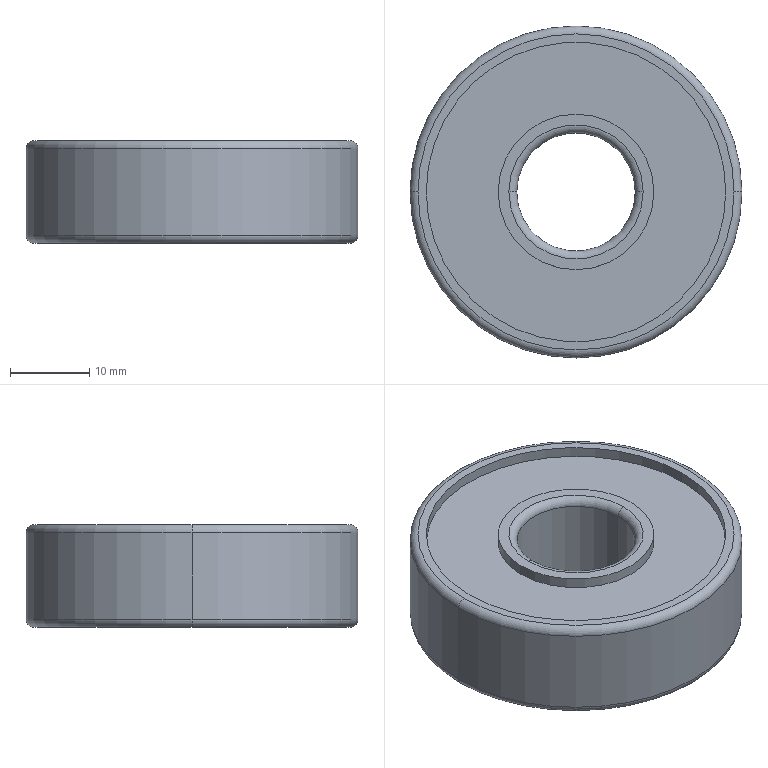Component | SolidWorks | Roller-01-2-1_B6302ZZ-2-1 | 1 solid | 26 faces | box 42 x 42 x 13 mm | volume 13427 mm3 | cylinder 12 | torus 8 | plane 6 | commonest cylinder face diameters 37.9 x4 19.7 x4 42 x2 15 x2
build123d program:
from build123d import *


with BuildPart() as part:
    # Sketch1 → Revolve1 (revolve)
    with BuildSketch(Plane.XY, mode=Mode.PRIVATE) as revolve1_sk:
        with BuildLine():
            Line((0, 20), (0, 18.95))
            Line((0, 18.95), (1.342, 18.95))
            Line((1.342, 18.95), (1.342, 9.85))
            Line((1.342, 9.85), (0, 9.85))
            Line((0, 9.85), (0, 8.5))
            ThreePointArc((0, 8.5), (0.2929, 7.793), (1, 7.5))
            Line((1, 7.5), (12, 7.5))
            ThreePointArc((12, 7.5), (12.707, 7.793), (13, 8.5))
            Line((13, 8.5), (13, 9.85))
            Line((13, 9.85), (11.658, 9.85))
            Line((11.658, 9.85), (11.658, 18.95))
            Line((11.658, 18.95), (13, 18.95))
            Line((13, 18.95), (13, 20))
            ThreePointArc((13, 20), (12.707, 20.707), (12, 21))
            Line((12, 21), (1, 21))
            ThreePointArc((1, 21), (0.2929, 20.707), (0, 20))
        make_face()
    revolve(revolve1_sk.sketch.rotate(Axis((13, 0, 0), (-1, 0, 0)), 270), axis=Axis((13, 0, 0), (-1, 0, 0)))


solid = part.part

# Placed as in the assembly
solid = solid.moved(Location((444.783, 71.385, -23.5), (0, 90, 0)))
STEP:
#1=COLOUR_RGB('',0.7922,0.8196,0.9333);
#2=FILL_AREA_STYLE_COLOUR('',#1);
#3=FILL_AREA_STYLE('',(#2));
#4=SURFACE_STYLE_FILL_AREA(#3);
#5=SURFACE_SIDE_STYLE('',(#4));
#6=SURFACE_STYLE_USAGE(.BOTH.,#5);
#7=PRESENTATION_STYLE_ASSIGNMENT((#6));
#8=CARTESIAN_POINT('',(18.338,2.81,-1.398));
#9=VERTEX_POINT('',#8);
#10=CARTESIAN_POINT('',(16.684,2.81,-1.398));
#11=VERTEX_POINT('',#10);
#12=CARTESIAN_POINT('',(17.511,2.81,-1.398));
#13=DIRECTION('',(0.,0.,1.));
#14=DIRECTION('',(1.,0.,0.));
#15=AXIS2_PLACEMENT_3D('',#12,#13,#14);
#16=CIRCLE('',#15,0.8268);
#17=EDGE_CURVE('',#9,#11,#16,.T.);
#18=ORIENTED_EDGE('',*,*,#17,.T.);
#19=CARTESIAN_POINT('',(16.684,2.81,-0.9646));
#20=VERTEX_POINT('',#19);
#21=CARTESIAN_POINT('',(16.684,2.81,-1.437));
#22=DIRECTION('',(0.,0.,1.));
#23=VECTOR('',#22,39.37);
#24=LINE('',#21,#23);
#25=EDGE_CURVE('',#11,#20,#24,.T.);
#26=ORIENTED_EDGE('',*,*,#25,.T.);
#27=CARTESIAN_POINT('',(18.338,2.81,-0.9646));
#28=VERTEX_POINT('',#27);
#29=CARTESIAN_POINT('',(17.511,2.81,-0.9646));
#30=DIRECTION('',(0.,0.,1.));
#31=DIRECTION('',(1.,0.,0.));
#32=AXIS2_PLACEMENT_3D('',#29,#30,#31);
#33=CIRCLE('',#32,0.8268);
#34=EDGE_CURVE('',#28,#20,#33,.T.);
#35=ORIENTED_EDGE('',*,*,#34,.F.);
#36=CARTESIAN_POINT('',(18.338,2.81,-1.437));
#37=DIRECTION('',(0.,0.,1.));
#38=VECTOR('',#37,39.37);
#39=LINE('',#36,#38);
#40=EDGE_CURVE('',#9,#28,#39,.T.);
#41=ORIENTED_EDGE('',*,*,#40,.F.);
#42=EDGE_LOOP('',(#18,#26,#35,#41));
#43=FACE_OUTER_BOUND('',#42,.T.);
#44=CARTESIAN_POINT('',(17.511,2.81,-1.437));
#45=DIRECTION('',(0.,0.,1.));
#46=DIRECTION('',(1.,0.,0.));
#47=AXIS2_PLACEMENT_3D('',#44,#45,#46);
#48=CYLINDRICAL_SURFACE('',#47,0.8268);
#49=ADVANCED_FACE('',(#43),#48,.T.);
#50=CARTESIAN_POINT('',(18.299,2.81,-1.437));
#51=VERTEX_POINT('',#50);
#52=CARTESIAN_POINT('',(16.724,2.81,-1.437));
#53=VERTEX_POINT('',#52);
#54=CARTESIAN_POINT('',(17.511,2.81,-1.437));
#55=DIRECTION('',(0.,0.,1.));
#56=DIRECTION('',(1.,0.,0.));
#57=AXIS2_PLACEMENT_3D('',#54,#55,#56);
#58=CIRCLE('',#57,0.7874);
#59=EDGE_CURVE('',#51,#53,#58,.T.);
#60=ORIENTED_EDGE('',*,*,#59,.T.);
#61=CARTESIAN_POINT('',(16.724,2.81,-1.398));
#62=DIRECTION('',(0.,1.,0.));
#63=DIRECTION('',(-1.,0.,0.));
#64=AXIS2_PLACEMENT_3D('',#61,#62,#63);
#65=CIRCLE('',#64,0.03937);
#66=EDGE_CURVE('',#53,#11,#65,.T.);
#67=ORIENTED_EDGE('',*,*,#66,.T.);
#68=ORIENTED_EDGE('',*,*,#17,.F.);
#69=CARTESIAN_POINT('',(18.299,2.81,-1.398));
#70=DIRECTION('',(0.,-1.,0.));
#71=DIRECTION('',(0.,0.,-1.));
#72=AXIS2_PLACEMENT_3D('',#69,#70,#71);
#73=CIRCLE('',#72,0.03937);
#74=EDGE_CURVE('',#51,#9,#73,.T.);
#75=ORIENTED_EDGE('',*,*,#74,.F.);
#76=EDGE_LOOP('',(#60,#67,#68,#75));
#77=FACE_OUTER_BOUND('',#76,.T.);
#78=CARTESIAN_POINT('',(17.511,2.81,-1.398));
#79=DIRECTION('',(0.,0.,1.));
#80=DIRECTION('',(1.,0.,0.));
#81=AXIS2_PLACEMENT_3D('',#78,#79,#80);
#82=TOROIDAL_SURFACE('',#81,0.7874,0.03937);
#83=ADVANCED_FACE('',(#77),#82,.T.);
#84=CARTESIAN_POINT('',(16.765,2.81,-1.437));
#85=VERTEX_POINT('',#84);
#86=CARTESIAN_POINT('',(18.257,2.81,-1.437));
#87=VERTEX_POINT('',#86);
#88=CARTESIAN_POINT('',(17.511,2.81,-1.437));
#89=DIRECTION('',(0.,0.,1.));
#90=DIRECTION('',(1.,0.,0.));
#91=AXIS2_PLACEMENT_3D('',#88,#89,#90);
#92=CIRCLE('',#91,0.7461);
#93=EDGE_CURVE('',#85,#87,#92,.T.);
#94=ORIENTED_EDGE('',*,*,#93,.F.);
#95=CARTESIAN_POINT('',(16.765,2.81,-1.384));
#96=VERTEX_POINT('',#95);
#97=CARTESIAN_POINT('',(16.765,2.81,-1.437));
#98=DIRECTION('',(0.,0.,1.));
#99=VECTOR('',#98,39.37);
#100=LINE('',#97,#99);
#101=EDGE_CURVE('',#85,#96,#100,.T.);
#102=ORIENTED_EDGE('',*,*,#101,.T.);
#103=CARTESIAN_POINT('',(18.257,2.81,-1.384));
#104=VERTEX_POINT('',#103);
#105=CARTESIAN_POINT('',(17.511,2.81,-1.384));
#106=DIRECTION('',(0.,0.,1.));
#107=DIRECTION('',(1.,0.,0.));
#108=AXIS2_PLACEMENT_3D('',#105,#106,#107);
#109=CIRCLE('',#108,0.7461);
#110=EDGE_CURVE('',#96,#104,#109,.T.);
#111=ORIENTED_EDGE('',*,*,#110,.T.);
#112=CARTESIAN_POINT('',(18.257,2.81,-1.437));
#113=DIRECTION('',(0.,0.,1.));
#114=VECTOR('',#113,39.37);
#115=LINE('',#112,#114);
#116=EDGE_CURVE('',#87,#104,#115,.T.);
#117=ORIENTED_EDGE('',*,*,#116,.F.);
#118=EDGE_LOOP('',(#94,#102,#111,#117));
#119=FACE_OUTER_BOUND('',#118,.T.);
#120=CARTESIAN_POINT('',(17.511,2.81,-1.437));
#121=DIRECTION('',(0.,0.,1.));
#122=DIRECTION('',(1.,0.,0.));
#123=AXIS2_PLACEMENT_3D('',#120,#121,#122);
#124=CYLINDRICAL_SURFACE('',#123,0.7461);
#125=ADVANCED_FACE('',(#119),#124,.F.);
#126=CARTESIAN_POINT('',(17.899,2.81,-1.437));
#127=VERTEX_POINT('',#126);
#128=CARTESIAN_POINT('',(17.123,2.81,-1.437));
#129=VERTEX_POINT('',#128);
#130=CARTESIAN_POINT('',(17.511,2.81,-1.437));
#131=DIRECTION('',(0.,0.,1.));
#132=DIRECTION('',(1.,0.,0.));
#133=AXIS2_PLACEMENT_3D('',#130,#131,#132);
#134=CIRCLE('',#133,0.3878);
#135=EDGE_CURVE('',#127,#129,#134,.T.);
#136=ORIENTED_EDGE('',*,*,#135,.T.);
#137=CARTESIAN_POINT('',(17.123,2.81,-1.384));
#138=VERTEX_POINT('',#137);
#139=CARTESIAN_POINT('',(17.123,2.81,-1.437));
#140=DIRECTION('',(0.,0.,1.));
#141=VECTOR('',#140,39.37);
#142=LINE('',#139,#141);
#143=EDGE_CURVE('',#129,#138,#142,.T.);
#144=ORIENTED_EDGE('',*,*,#143,.T.);
#145=CARTESIAN_POINT('',(17.899,2.81,-1.384));
#146=VERTEX_POINT('',#145);
#147=CARTESIAN_POINT('',(17.511,2.81,-1.384));
#148=DIRECTION('',(0.,0.,1.));
#149=DIRECTION('',(1.,0.,0.));
#150=AXIS2_PLACEMENT_3D('',#147,#148,#149);
#151=CIRCLE('',#150,0.3878);
#152=EDGE_CURVE('',#146,#138,#151,.T.);
#153=ORIENTED_EDGE('',*,*,#152,.F.);
#154=CARTESIAN_POINT('',(17.899,2.81,-1.437));
#155=DIRECTION('',(0.,0.,1.));
#156=VECTOR('',#155,39.37);
#157=LINE('',#154,#156);
#158=EDGE_CURVE('',#127,#146,#157,.T.);
#159=ORIENTED_EDGE('',*,*,#158,.F.);
#160=EDGE_LOOP('',(#136,#144,#153,#159));
#161=FACE_OUTER_BOUND('',#160,.T.);
#162=CARTESIAN_POINT('',(17.511,2.81,-1.437));
#163=DIRECTION('',(0.,0.,1.));
#164=DIRECTION('',(1.,0.,0.));
#165=AXIS2_PLACEMENT_3D('',#162,#163,#164);
#166=CYLINDRICAL_SURFACE('',#165,0.3878);
#167=ADVANCED_FACE('',(#161),#166,.T.);
#168=CARTESIAN_POINT('',(17.806,2.81,-1.398));
#169=VERTEX_POINT('',#168);
#170=CARTESIAN_POINT('',(17.216,2.81,-1.398));
#171=VERTEX_POINT('',#170);
#172=CARTESIAN_POINT('',(17.511,2.81,-1.398));
#173=DIRECTION('',(0.,0.,1.));
#174=DIRECTION('',(1.,0.,0.));
#175=AXIS2_PLACEMENT_3D('',#172,#173,#174);
#176=CIRCLE('',#175,0.2953);
#177=EDGE_CURVE('',#169,#171,#176,.T.);
#178=ORIENTED_EDGE('',*,*,#177,.T.);
#179=CARTESIAN_POINT('',(17.177,2.81,-1.437));
#180=VERTEX_POINT('',#179);
#181=CARTESIAN_POINT('',(17.177,2.81,-1.398));
#182=DIRECTION('',(0.,1.,0.));
#183=DIRECTION('',(-1.,0.,0.));
#184=AXIS2_PLACEMENT_3D('',#181,#182,#183);
#185=CIRCLE('',#184,0.03937);
#186=EDGE_CURVE('',#171,#180,#185,.T.);
#187=ORIENTED_EDGE('',*,*,#186,.T.);
#188=CARTESIAN_POINT('',(17.846,2.81,-1.437));
#189=VERTEX_POINT('',#188);
#190=CARTESIAN_POINT('',(17.511,2.81,-1.437));
#191=DIRECTION('',(0.,0.,1.));
#192=DIRECTION('',(1.,0.,0.));
#193=AXIS2_PLACEMENT_3D('',#190,#191,#192);
#194=CIRCLE('',#193,0.3346);
#195=EDGE_CURVE('',#189,#180,#194,.T.);
#196=ORIENTED_EDGE('',*,*,#195,.F.);
#197=CARTESIAN_POINT('',(17.846,2.81,-1.398));
#198=DIRECTION('',(0.,-1.,0.));
#199=DIRECTION('',(0.,0.,-1.));
#200=AXIS2_PLACEMENT_3D('',#197,#198,#199);
#201=CIRCLE('',#200,0.03937);
#202=EDGE_CURVE('',#169,#189,#201,.T.);
#203=ORIENTED_EDGE('',*,*,#202,.F.);
#204=EDGE_LOOP('',(#178,#187,#196,#203));
#205=FACE_OUTER_BOUND('',#204,.T.);
#206=CARTESIAN_POINT('',(17.511,2.81,-1.398));
#207=DIRECTION('',(0.,0.,1.));
#208=DIRECTION('',(1.,0.,0.));
#209=AXIS2_PLACEMENT_3D('',#206,#207,#208);
#210=TOROIDAL_SURFACE('',#209,0.3346,0.03937);
#211=ADVANCED_FACE('',(#205),#210,.T.);
#212=CARTESIAN_POINT('',(17.511,2.81,-1.398));
#213=DIRECTION('',(0.,0.,1.));
#214=DIRECTION('',(1.,0.,0.));
#215=AXIS2_PLACEMENT_3D('',#212,#213,#214);
#216=CIRCLE('',#215,0.2953);
#217=EDGE_CURVE('',#171,#169,#216,.T.);
#218=ORIENTED_EDGE('',*,*,#217,.F.);
#219=CARTESIAN_POINT('',(17.216,2.81,-0.9646));
#220=VERTEX_POINT('',#219);
#221=CARTESIAN_POINT('',(17.216,2.81,-1.437));
#222=DIRECTION('',(0.,0.,1.));
#223=VECTOR('',#222,39.37);
#224=LINE('',#221,#223);
#225=EDGE_CURVE('',#171,#220,#224,.T.);
#226=ORIENTED_EDGE('',*,*,#225,.T.);
#227=CARTESIAN_POINT('',(17.806,2.81,-0.9646));
#228=VERTEX_POINT('',#227);
#229=CARTESIAN_POINT('',(17.511,2.81,-0.9646));
#230=DIRECTION('',(0.,0.,1.));
#231=DIRECTION('',(1.,0.,0.));
#232=AXIS2_PLACEMENT_3D('',#229,#230,#231);
#233=CIRCLE('',#232,0.2953);
#234=EDGE_CURVE('',#220,#228,#233,.T.);
#235=ORIENTED_EDGE('',*,*,#234,.T.);
#236=CARTESIAN_POINT('',(17.806,2.81,-1.437));
#237=DIRECTION('',(0.,0.,1.));
#238=VECTOR('',#237,39.37);
#239=LINE('',#236,#238);
#240=EDGE_CURVE('',#169,#228,#239,.T.);
#241=ORIENTED_EDGE('',*,*,#240,.F.);
#242=EDGE_LOOP('',(#218,#226,#235,#241));
#243=FACE_OUTER_BOUND('',#242,.T.);
#244=CARTESIAN_POINT('',(17.511,2.81,-1.437));
#245=DIRECTION('',(0.,0.,1.));
#246=DIRECTION('',(1.,0.,0.));
#247=AXIS2_PLACEMENT_3D('',#244,#245,#246);
#248=CYLINDRICAL_SURFACE('',#247,0.2953);
#249=ADVANCED_FACE('',(#243),#248,.F.);
#250=CARTESIAN_POINT('',(17.846,2.81,-0.9252));
#251=VERTEX_POINT('',#250);
#252=CARTESIAN_POINT('',(17.177,2.81,-0.9252));
#253=VERTEX_POINT('',#252);
#254=CARTESIAN_POINT('',(17.511,2.81,-0.9252));
#255=DIRECTION('',(0.,0.,1.));
#256=DIRECTION('',(1.,0.,0.));
#257=AXIS2_PLACEMENT_3D('',#254,#255,#256);
#258=CIRCLE('',#257,0.3346);
#259=EDGE_CURVE('',#251,#253,#258,.T.);
#260=ORIENTED_EDGE('',*,*,#259,.T.);
#261=CARTESIAN_POINT('',(17.177,2.81,-0.9646));
#262=DIRECTION('',(0.,1.,0.));
#263=DIRECTION('',(-1.,0.,0.));
#264=AXIS2_PLACEMENT_3D('',#261,#262,#263);
#265=CIRCLE('',#264,0.03937);
#266=EDGE_CURVE('',#253,#220,#265,.T.);
#267=ORIENTED_EDGE('',*,*,#266,.T.);
#268=CARTESIAN_POINT('',(17.511,2.81,-0.9646));
#269=DIRECTION('',(0.,0.,1.));
#270=DIRECTION('',(1.,0.,0.));
#271=AXIS2_PLACEMENT_3D('',#268,#269,#270);
#272=CIRCLE('',#271,0.2953);
#273=EDGE_CURVE('',#228,#220,#272,.T.);
#274=ORIENTED_EDGE('',*,*,#273,.F.);
#275=CARTESIAN_POINT('',(17.846,2.81,-0.9646));
#276=DIRECTION('',(0.,-1.,0.));
#277=DIRECTION('',(0.,0.,-1.));
#278=AXIS2_PLACEMENT_3D('',#275,#276,#277);
#279=CIRCLE('',#278,0.03937);
#280=EDGE_CURVE('',#251,#228,#279,.T.);
#281=ORIENTED_EDGE('',*,*,#280,.F.);
#282=EDGE_LOOP('',(#260,#267,#274,#281));
#283=FACE_OUTER_BOUND('',#282,.T.);
#284=CARTESIAN_POINT('',(17.511,2.81,-0.9646));
#285=DIRECTION('',(0.,0.,1.));
#286=DIRECTION('',(1.,0.,0.));
#287=AXIS2_PLACEMENT_3D('',#284,#285,#286);
#288=TOROIDAL_SURFACE('',#287,0.3346,0.03937);
#289=ADVANCED_FACE('',(#283),#288,.T.);
#290=CARTESIAN_POINT('',(17.899,2.81,-0.978));
#291=VERTEX_POINT('',#290);
#292=CARTESIAN_POINT('',(17.123,2.81,-0.978));
#293=VERTEX_POINT('',#292);
#294=CARTESIAN_POINT('',(17.511,2.81,-0.978));
#295=DIRECTION('',(0.,0.,1.));
#296=DIRECTION('',(1.,0.,0.));
#297=AXIS2_PLACEMENT_3D('',#294,#295,#296);
#298=CIRCLE('',#297,0.3878);
#299=EDGE_CURVE('',#291,#293,#298,.T.);
#300=ORIENTED_EDGE('',*,*,#299,.T.);
#301=CARTESIAN_POINT('',(17.123,2.81,-0.9252));
#302=VERTEX_POINT('',#301);
#303=CARTESIAN_POINT('',(17.123,2.81,-1.437));
#304=DIRECTION('',(0.,0.,1.));
#305=VECTOR('',#304,39.37);
#306=LINE('',#303,#305);
#307=EDGE_CURVE('',#293,#302,#306,.T.);
#308=ORIENTED_EDGE('',*,*,#307,.T.);
#309=CARTESIAN_POINT('',(17.899,2.81,-0.9252));
#310=VERTEX_POINT('',#309);
#311=CARTESIAN_POINT('',(17.511,2.81,-0.9252));
#312=DIRECTION('',(0.,0.,1.));
#313=DIRECTION('',(1.,0.,0.));
#314=AXIS2_PLACEMENT_3D('',#311,#312,#313);
#315=CIRCLE('',#314,0.3878);
#316=EDGE_CURVE('',#310,#302,#315,.T.);
#317=ORIENTED_EDGE('',*,*,#316,.F.);
#318=CARTESIAN_POINT('',(17.899,2.81,-1.437));
#319=DIRECTION('',(0.,0.,1.));
#320=VECTOR('',#319,39.37);
#321=LINE('',#318,#320);
#322=EDGE_CURVE('',#291,#310,#321,.T.);
#323=ORIENTED_EDGE('',*,*,#322,.F.);
#324=EDGE_LOOP('',(#300,#308,#317,#323));
#325=FACE_OUTER_BOUND('',#324,.T.);
#326=CARTESIAN_POINT('',(17.511,2.81,-1.437));
#327=DIRECTION('',(0.,0.,1.));
#328=DIRECTION('',(1.,0.,0.));
#329=AXIS2_PLACEMENT_3D('',#326,#327,#328);
#330=CYLINDRICAL_SURFACE('',#329,0.3878);
#331=ADVANCED_FACE('',(#325),#330,.T.);
#332=CARTESIAN_POINT('',(16.765,2.81,-0.978));
#333=VERTEX_POINT('',#332);
#334=CARTESIAN_POINT('',(18.257,2.81,-0.978));
#335=VERTEX_POINT('',#334);
#336=CARTESIAN_POINT('',(17.511,2.81,-0.978));
#337=DIRECTION('',(0.,0.,1.));
#338=DIRECTION('',(1.,0.,0.));
#339=AXIS2_PLACEMENT_3D('',#336,#337,#338);
#340=CIRCLE('',#339,0.7461);
#341=EDGE_CURVE('',#333,#335,#340,.T.);
#342=ORIENTED_EDGE('',*,*,#341,.F.);
#343=CARTESIAN_POINT('',(16.765,2.81,-0.9252));
#344=VERTEX_POINT('',#343);
#345=CARTESIAN_POINT('',(16.765,2.81,-1.437));
#346=DIRECTION('',(0.,0.,1.));
#347=VECTOR('',#346,39.37);
#348=LINE('',#345,#347);
#349=EDGE_CURVE('',#333,#344,#348,.T.);
#350=ORIENTED_EDGE('',*,*,#349,.T.);
#351=CARTESIAN_POINT('',(18.257,2.81,-0.9252));
#352=VERTEX_POINT('',#351);
#353=CARTESIAN_POINT('',(17.511,2.81,-0.9252));
#354=DIRECTION('',(0.,0.,1.));
#355=DIRECTION('',(1.,0.,0.));
#356=AXIS2_PLACEMENT_3D('',#353,#354,#355);
#357=CIRCLE('',#356,0.7461);
#358=EDGE_CURVE('',#344,#352,#357,.T.);
#359=ORIENTED_EDGE('',*,*,#358,.T.);
#360=CARTESIAN_POINT('',(18.257,2.81,-1.437));
#361=DIRECTION('',(0.,0.,1.));
#362=VECTOR('',#361,39.37);
#363=LINE('',#360,#362);
#364=EDGE_CURVE('',#335,#352,#363,.T.);
#365=ORIENTED_EDGE('',*,*,#364,.F.);
#366=EDGE_LOOP('',(#342,#350,#359,#365));
#367=FACE_OUTER_BOUND('',#366,.T.);
#368=CARTESIAN_POINT('',(17.511,2.81,-1.437));
#369=DIRECTION('',(0.,0.,1.));
#370=DIRECTION('',(1.,0.,0.));
#371=AXIS2_PLACEMENT_3D('',#368,#369,#370);
#372=CYLINDRICAL_SURFACE('',#371,0.7461);
#373=ADVANCED_FACE('',(#367),#372,.F.);
#374=ORIENTED_EDGE('',*,*,#34,.T.);
#375=CARTESIAN_POINT('',(16.724,2.81,-0.9252));
#376=VERTEX_POINT('',#375);
#377=CARTESIAN_POINT('',(16.724,2.81,-0.9646));
#378=DIRECTION('',(0.,1.,0.));
#379=DIRECTION('',(-1.,0.,0.));
#380=AXIS2_PLACEMENT_3D('',#377,#378,#379);
#381=CIRCLE('',#380,0.03937);
#382=EDGE_CURVE('',#20,#376,#381,.T.);
#383=ORIENTED_EDGE('',*,*,#382,.T.);
#384=CARTESIAN_POINT('',(18.299,2.81,-0.9252));
#385=VERTEX_POINT('',#384);
#386=CARTESIAN_POINT('',(17.511,2.81,-0.9252));
#387=DIRECTION('',(0.,0.,1.));
#388=DIRECTION('',(1.,0.,0.));
#389=AXIS2_PLACEMENT_3D('',#386,#387,#388);
#390=CIRCLE('',#389,0.7874);
#391=EDGE_CURVE('',#385,#376,#390,.T.);
#392=ORIENTED_EDGE('',*,*,#391,.F.);
#393=CARTESIAN_POINT('',(18.299,2.81,-0.9646));
#394=DIRECTION('',(0.,-1.,0.));
#395=DIRECTION('',(0.,0.,-1.));
#396=AXIS2_PLACEMENT_3D('',#393,#394,#395);
#397=CIRCLE('',#396,0.03937);
#398=EDGE_CURVE('',#28,#385,#397,.T.);
#399=ORIENTED_EDGE('',*,*,#398,.F.);
#400=EDGE_LOOP('',(#374,#383,#392,#399));
#401=FACE_OUTER_BOUND('',#400,.T.);
#402=CARTESIAN_POINT('',(17.511,2.81,-0.9646));
#403=DIRECTION('',(0.,0.,1.));
#404=DIRECTION('',(1.,0.,0.));
#405=AXIS2_PLACEMENT_3D('',#402,#403,#404);
#406=TOROIDAL_SURFACE('',#405,0.7874,0.03937);
#407=ADVANCED_FACE('',(#401),#406,.T.);
#408=ORIENTED_EDGE('',*,*,#382,.F.);
#409=CARTESIAN_POINT('',(17.511,2.81,-0.9646));
#410=DIRECTION('',(0.,0.,1.));
#411=DIRECTION('',(1.,0.,0.));
#412=AXIS2_PLACEMENT_3D('',#409,#410,#411);
#413=CIRCLE('',#412,0.8268);
#414=EDGE_CURVE('',#20,#28,#413,.T.);
#415=ORIENTED_EDGE('',*,*,#414,.T.);
#416=ORIENTED_EDGE('',*,*,#398,.T.);
#417=CARTESIAN_POINT('',(17.511,2.81,-0.9252));
#418=DIRECTION('',(0.,0.,1.));
#419=DIRECTION('',(1.,0.,0.));
#420=AXIS2_PLACEMENT_3D('',#417,#418,#419);
#421=CIRCLE('',#420,0.7874);
#422=EDGE_CURVE('',#376,#385,#421,.T.);
#423=ORIENTED_EDGE('',*,*,#422,.F.);
#424=EDGE_LOOP('',(#408,#415,#416,#423));
#425=FACE_OUTER_BOUND('',#424,.T.);
#426=CARTESIAN_POINT('',(17.511,2.81,-0.9646));
#427=DIRECTION('',(0.,0.,1.));
#428=DIRECTION('',(1.,0.,0.));
#429=AXIS2_PLACEMENT_3D('',#426,#427,#428);
#430=TOROIDAL_SURFACE('',#429,0.7874,0.03937);
#431=ADVANCED_FACE('',(#425),#430,.T.);
#432=CARTESIAN_POINT('',(17.511,2.81,-0.9252));
#433=DIRECTION('',(0.,0.,1.));
#434=DIRECTION('',(1.,0.,0.));
#435=AXIS2_PLACEMENT_3D('',#432,#433,#434);
#436=CIRCLE('',#435,0.7461);
#437=EDGE_CURVE('',#352,#344,#436,.T.);
#438=ORIENTED_EDGE('',*,*,#437,.F.);
#439=ORIENTED_EDGE('',*,*,#358,.F.);
#440=EDGE_LOOP('',(#438,#439));
#441=FACE_BOUND('',#440,.T.);
#442=ORIENTED_EDGE('',*,*,#391,.T.);
#443=ORIENTED_EDGE('',*,*,#422,.T.);
#444=EDGE_LOOP('',(#442,#443));
#445=FACE_OUTER_BOUND('',#444,.T.);
#446=CARTESIAN_POINT('',(17.511,3.598,-0.9252));
#447=DIRECTION('',(0.,0.,-1.));
#448=DIRECTION('',(-1.,0.,0.));
#449=AXIS2_PLACEMENT_3D('',#446,#447,#448);
#450=PLANE('',#449);
#451=ADVANCED_FACE('',(#441,#445),#450,.F.);
#452=ORIENTED_EDGE('',*,*,#349,.F.);
#453=CARTESIAN_POINT('',(17.511,2.81,-0.978));
#454=DIRECTION('',(0.,0.,1.));
#455=DIRECTION('',(1.,0.,0.));
#456=AXIS2_PLACEMENT_3D('',#453,#454,#455);
#457=CIRCLE('',#456,0.7461);
#458=EDGE_CURVE('',#335,#333,#457,.T.);
#459=ORIENTED_EDGE('',*,*,#458,.F.);
#460=ORIENTED_EDGE('',*,*,#364,.T.);
#461=ORIENTED_EDGE('',*,*,#437,.T.);
#462=EDGE_LOOP('',(#452,#459,#460,#461));
#463=FACE_OUTER_BOUND('',#462,.T.);
#464=CARTESIAN_POINT('',(17.511,2.81,-1.437));
#465=DIRECTION('',(0.,0.,1.));
#466=DIRECTION('',(1.,0.,0.));
#467=AXIS2_PLACEMENT_3D('',#464,#465,#466);
#468=CYLINDRICAL_SURFACE('',#467,0.7461);
#469=ADVANCED_FACE('',(#463),#468,.F.);
#470=ORIENTED_EDGE('',*,*,#299,.F.);
#471=CARTESIAN_POINT('',(17.511,2.81,-0.978));
#472=DIRECTION('',(0.,0.,1.));
#473=DIRECTION('',(1.,0.,0.));
#474=AXIS2_PLACEMENT_3D('',#471,#472,#473);
#475=CIRCLE('',#474,0.3878);
#476=EDGE_CURVE('',#293,#291,#475,.T.);
#477=ORIENTED_EDGE('',*,*,#476,.F.);
#478=EDGE_LOOP('',(#470,#477));
#479=FACE_BOUND('',#478,.T.);
#480=ORIENTED_EDGE('',*,*,#458,.T.);
#481=ORIENTED_EDGE('',*,*,#341,.T.);
#482=EDGE_LOOP('',(#480,#481));
#483=FACE_OUTER_BOUND('',#482,.T.);
#484=CARTESIAN_POINT('',(17.511,3.556,-0.978));
#485=DIRECTION('',(0.,0.,-1.));
#486=DIRECTION('',(-1.,0.,0.));
#487=AXIS2_PLACEMENT_3D('',#484,#485,#486);
#488=PLANE('',#487);
#489=ADVANCED_FACE('',(#479,#483),#488,.F.);
#490=ORIENTED_EDGE('',*,*,#307,.F.);
#491=ORIENTED_EDGE('',*,*,#476,.T.);
#492=ORIENTED_EDGE('',*,*,#322,.T.);
#493=CARTESIAN_POINT('',(17.511,2.81,-0.9252));
#494=DIRECTION('',(0.,0.,1.));
#495=DIRECTION('',(1.,0.,0.));
#496=AXIS2_PLACEMENT_3D('',#493,#494,#495);
#497=CIRCLE('',#496,0.3878);
#498=EDGE_CURVE('',#302,#310,#497,.T.);
#499=ORIENTED_EDGE('',*,*,#498,.F.);
#500=EDGE_LOOP('',(#490,#491,#492,#499));
#501=FACE_OUTER_BOUND('',#500,.T.);
#502=CARTESIAN_POINT('',(17.511,2.81,-1.437));
#503=DIRECTION('',(0.,0.,1.));
#504=DIRECTION('',(1.,0.,0.));
#505=AXIS2_PLACEMENT_3D('',#502,#503,#504);
#506=CYLINDRICAL_SURFACE('',#505,0.3878);
#507=ADVANCED_FACE('',(#501),#506,.T.);
#508=ORIENTED_EDGE('',*,*,#259,.F.);
#509=CARTESIAN_POINT('',(17.511,2.81,-0.9252));
#510=DIRECTION('',(0.,0.,1.));
#511=DIRECTION('',(1.,0.,0.));
#512=AXIS2_PLACEMENT_3D('',#509,#510,#511);
#513=CIRCLE('',#512,0.3346);
#514=EDGE_CURVE('',#253,#251,#513,.T.);
#515=ORIENTED_EDGE('',*,*,#514,.F.);
#516=EDGE_LOOP('',(#508,#515));
#517=FACE_BOUND('',#516,.T.);
#518=ORIENTED_EDGE('',*,*,#316,.T.);
#519=ORIENTED_EDGE('',*,*,#498,.T.);
#520=EDGE_LOOP('',(#518,#519));
#521=FACE_OUTER_BOUND('',#520,.T.);
#522=CARTESIAN_POINT('',(17.511,3.198,-0.9252));
#523=DIRECTION('',(0.,0.,-1.));
#524=DIRECTION('',(-1.,0.,0.));
#525=AXIS2_PLACEMENT_3D('',#522,#523,#524);
#526=PLANE('',#525);
#527=ADVANCED_FACE('',(#517,#521),#526,.F.);
#528=ORIENTED_EDGE('',*,*,#266,.F.);
#529=ORIENTED_EDGE('',*,*,#514,.T.);
#530=ORIENTED_EDGE('',*,*,#280,.T.);
#531=ORIENTED_EDGE('',*,*,#234,.F.);
#532=EDGE_LOOP('',(#528,#529,#530,#531));
#533=FACE_OUTER_BOUND('',#532,.T.);
#534=CARTESIAN_POINT('',(17.511,2.81,-0.9646));
#535=DIRECTION('',(0.,0.,1.));
#536=DIRECTION('',(1.,0.,0.));
#537=AXIS2_PLACEMENT_3D('',#534,#535,#536);
#538=TOROIDAL_SURFACE('',#537,0.3346,0.03937);
#539=ADVANCED_FACE('',(#533),#538,.T.);
#540=ORIENTED_EDGE('',*,*,#225,.F.);
#541=ORIENTED_EDGE('',*,*,#177,.F.);
#542=ORIENTED_EDGE('',*,*,#240,.T.);
#543=ORIENTED_EDGE('',*,*,#273,.T.);
#544=EDGE_LOOP('',(#540,#541,#542,#543));
#545=FACE_OUTER_BOUND('',#544,.T.);
#546=CARTESIAN_POINT('',(17.511,2.81,-1.437));
#547=DIRECTION('',(0.,0.,1.));
#548=DIRECTION('',(1.,0.,0.));
#549=AXIS2_PLACEMENT_3D('',#546,#547,#548);
#550=CYLINDRICAL_SURFACE('',#549,0.2953);
#551=ADVANCED_FACE('',(#545),#550,.F.);
#552=ORIENTED_EDGE('',*,*,#186,.F.);
#553=ORIENTED_EDGE('',*,*,#217,.T.);
#554=ORIENTED_EDGE('',*,*,#202,.T.);
#555=CARTESIAN_POINT('',(17.511,2.81,-1.437));
#556=DIRECTION('',(0.,0.,1.));
#557=DIRECTION('',(1.,0.,0.));
#558=AXIS2_PLACEMENT_3D('',#555,#556,#557);
#559=CIRCLE('',#558,0.3346);
#560=EDGE_CURVE('',#180,#189,#559,.T.);
#561=ORIENTED_EDGE('',*,*,#560,.F.);
#562=EDGE_LOOP('',(#552,#553,#554,#561));
#563=FACE_OUTER_BOUND('',#562,.T.);
#564=CARTESIAN_POINT('',(17.511,2.81,-1.398));
#565=DIRECTION('',(0.,0.,1.));
#566=DIRECTION('',(1.,0.,0.));
#567=AXIS2_PLACEMENT_3D('',#564,#565,#566);
#568=TOROIDAL_SURFACE('',#567,0.3346,0.03937);
#569=ADVANCED_FACE('',(#563),#568,.T.);
#570=ORIENTED_EDGE('',*,*,#135,.F.);
#571=CARTESIAN_POINT('',(17.511,2.81,-1.437));
#572=DIRECTION('',(0.,0.,1.));
#573=DIRECTION('',(1.,0.,0.));
#574=AXIS2_PLACEMENT_3D('',#571,#572,#573);
#575=CIRCLE('',#574,0.3878);
#576=EDGE_CURVE('',#129,#127,#575,.T.);
#577=ORIENTED_EDGE('',*,*,#576,.F.);
#578=EDGE_LOOP('',(#570,#577));
#579=FACE_OUTER_BOUND('',#578,.T.);
#580=ORIENTED_EDGE('',*,*,#195,.T.);
#581=ORIENTED_EDGE('',*,*,#560,.T.);
#582=EDGE_LOOP('',(#580,#581));
#583=FACE_BOUND('',#582,.T.);
#584=CARTESIAN_POINT('',(17.511,3.145,-1.437));
#585=DIRECTION('',(0.,0.,1.));
#586=DIRECTION('',(1.,0.,0.));
#587=AXIS2_PLACEMENT_3D('',#584,#585,#586);
#588=PLANE('',#587);
#589=ADVANCED_FACE('',(#579,#583),#588,.F.);
#590=ORIENTED_EDGE('',*,*,#143,.F.);
#591=ORIENTED_EDGE('',*,*,#576,.T.);
#592=ORIENTED_EDGE('',*,*,#158,.T.);
#593=CARTESIAN_POINT('',(17.511,2.81,-1.384));
#594=DIRECTION('',(0.,0.,1.));
#595=DIRECTION('',(1.,0.,0.));
#596=AXIS2_PLACEMENT_3D('',#593,#594,#595);
#597=CIRCLE('',#596,0.3878);
#598=EDGE_CURVE('',#138,#146,#597,.T.);
#599=ORIENTED_EDGE('',*,*,#598,.F.);
#600=EDGE_LOOP('',(#590,#591,#592,#599));
#601=FACE_OUTER_BOUND('',#600,.T.);
#602=CARTESIAN_POINT('',(17.511,2.81,-1.437));
#603=DIRECTION('',(0.,0.,1.));
#604=DIRECTION('',(1.,0.,0.));
#605=AXIS2_PLACEMENT_3D('',#602,#603,#604);
#606=CYLINDRICAL_SURFACE('',#605,0.3878);
#607=ADVANCED_FACE('',(#601),#606,.T.);
#608=CARTESIAN_POINT('',(17.511,2.81,-1.384));
#609=DIRECTION('',(0.,0.,1.));
#610=DIRECTION('',(1.,0.,0.));
#611=AXIS2_PLACEMENT_3D('',#608,#609,#610);
#612=CIRCLE('',#611,0.7461);
#613=EDGE_CURVE('',#104,#96,#612,.T.);
#614=ORIENTED_EDGE('',*,*,#613,.F.);
#615=ORIENTED_EDGE('',*,*,#110,.F.);
#616=EDGE_LOOP('',(#614,#615));
#617=FACE_OUTER_BOUND('',#616,.T.);
#618=ORIENTED_EDGE('',*,*,#152,.T.);
#619=ORIENTED_EDGE('',*,*,#598,.T.);
#620=EDGE_LOOP('',(#618,#619));
#621=FACE_BOUND('',#620,.T.);
#622=CARTESIAN_POINT('',(17.511,3.198,-1.384));
#623=DIRECTION('',(0.,0.,1.));
#624=DIRECTION('',(1.,0.,0.));
#625=AXIS2_PLACEMENT_3D('',#622,#623,#624);
#626=PLANE('',#625);
#627=ADVANCED_FACE('',(#617,#621),#626,.F.);
#628=ORIENTED_EDGE('',*,*,#101,.F.);
#629=CARTESIAN_POINT('',(17.511,2.81,-1.437));
#630=DIRECTION('',(0.,0.,1.));
#631=DIRECTION('',(1.,0.,0.));
#632=AXIS2_PLACEMENT_3D('',#629,#630,#631);
#633=CIRCLE('',#632,0.7461);
#634=EDGE_CURVE('',#87,#85,#633,.T.);
#635=ORIENTED_EDGE('',*,*,#634,.F.);
#636=ORIENTED_EDGE('',*,*,#116,.T.);
#637=ORIENTED_EDGE('',*,*,#613,.T.);
#638=EDGE_LOOP('',(#628,#635,#636,#637));
#639=FACE_OUTER_BOUND('',#638,.T.);
#640=CARTESIAN_POINT('',(17.511,2.81,-1.437));
#641=DIRECTION('',(0.,0.,1.));
#642=DIRECTION('',(1.,0.,0.));
#643=AXIS2_PLACEMENT_3D('',#640,#641,#642);
#644=CYLINDRICAL_SURFACE('',#643,0.7461);
#645=ADVANCED_FACE('',(#639),#644,.F.);
#646=ORIENTED_EDGE('',*,*,#59,.F.);
#647=CARTESIAN_POINT('',(17.511,2.81,-1.437));
#648=DIRECTION('',(0.,0.,1.));
#649=DIRECTION('',(1.,0.,0.));
#650=AXIS2_PLACEMENT_3D('',#647,#648,#649);
#651=CIRCLE('',#650,0.7874);
#652=EDGE_CURVE('',#53,#51,#651,.T.);
#653=ORIENTED_EDGE('',*,*,#652,.F.);
#654=EDGE_LOOP('',(#646,#653));
#655=FACE_OUTER_BOUND('',#654,.T.);
#656=ORIENTED_EDGE('',*,*,#634,.T.);
#657=ORIENTED_EDGE('',*,*,#93,.T.);
#658=EDGE_LOOP('',(#656,#657));
#659=FACE_BOUND('',#658,.T.);
#660=CARTESIAN_POINT('',(17.511,3.556,-1.437));
#661=DIRECTION('',(0.,0.,1.));
#662=DIRECTION('',(1.,0.,0.));
#663=AXIS2_PLACEMENT_3D('',#660,#661,#662);
#664=PLANE('',#663);
#665=ADVANCED_FACE('',(#655,#659),#664,.F.);
#666=ORIENTED_EDGE('',*,*,#66,.F.);
#667=ORIENTED_EDGE('',*,*,#652,.T.);
#668=ORIENTED_EDGE('',*,*,#74,.T.);
#669=CARTESIAN_POINT('',(17.511,2.81,-1.398));
#670=DIRECTION('',(0.,0.,1.));
#671=DIRECTION('',(1.,0.,0.));
#672=AXIS2_PLACEMENT_3D('',#669,#670,#671);
#673=CIRCLE('',#672,0.8268);
#674=EDGE_CURVE('',#11,#9,#673,.T.);
#675=ORIENTED_EDGE('',*,*,#674,.F.);
#676=EDGE_LOOP('',(#666,#667,#668,#675));
#677=FACE_OUTER_BOUND('',#676,.T.);
#678=CARTESIAN_POINT('',(17.511,2.81,-1.398));
#679=DIRECTION('',(0.,0.,1.));
#680=DIRECTION('',(1.,0.,0.));
#681=AXIS2_PLACEMENT_3D('',#678,#679,#680);
#682=TOROIDAL_SURFACE('',#681,0.7874,0.03937);
#683=ADVANCED_FACE('',(#677),#682,.T.);
#684=ORIENTED_EDGE('',*,*,#25,.F.);
#685=ORIENTED_EDGE('',*,*,#674,.T.);
#686=ORIENTED_EDGE('',*,*,#40,.T.);
#687=ORIENTED_EDGE('',*,*,#414,.F.);
#688=EDGE_LOOP('',(#684,#685,#686,#687));
#689=FACE_OUTER_BOUND('',#688,.T.);
#690=CARTESIAN_POINT('',(17.511,2.81,-1.437));
#691=DIRECTION('',(0.,0.,1.));
#692=DIRECTION('',(1.,0.,0.));
#693=AXIS2_PLACEMENT_3D('',#690,#691,#692);
#694=CYLINDRICAL_SURFACE('',#693,0.8268);
#695=ADVANCED_FACE('',(#689),#694,.T.);
#696=CLOSED_SHELL('',(#49,#83,#125,#167,#211,#249,#289,#331,#373,#407,#431,#451,#469,#489,#507,#527,#539,#551,#569,#589,#607,#627,#645,#665,#683,#695));
#697=MANIFOLD_SOLID_BREP('',#696);
#698=STYLED_ITEM('',(#7),#697);
#699=(LENGTH_UNIT()NAMED_UNIT(*)SI_UNIT($,.METRE.));
#700=LENGTH_MEASURE_WITH_UNIT(LENGTH_MEASURE(0.0254),#699);
#701=DIMENSIONAL_EXPONENTS(1.,0.,0.,0.,0.,0.,0.);
#702=(CONVERSION_BASED_UNIT('',#700)LENGTH_UNIT()NAMED_UNIT(#701));
#703=UNCERTAINTY_MEASURE_WITH_UNIT(LENGTH_MEASURE(0.00001),#702,'','');
#704=(NAMED_UNIT(*)PLANE_ANGLE_UNIT()SI_UNIT($,.RADIAN.));
#705=(NAMED_UNIT(*)SI_UNIT($,.STERADIAN.)SOLID_ANGLE_UNIT());
#706=(GEOMETRIC_REPRESENTATION_CONTEXT(3)GLOBAL_UNCERTAINTY_ASSIGNED_CONTEXT((#703))GLOBAL_UNIT_ASSIGNED_CONTEXT((#702,#704,#705))REPRESENTATION_CONTEXT('',''));
#707=MECHANICAL_DESIGN_GEOMETRIC_PRESENTATION_REPRESENTATION('',(#698),#706);
#708=CARTESIAN_POINT('',(0.,0.,0.));
#709=DIRECTION('',(0.,0.,1.));
#710=DIRECTION('',(1.,0.,0.));
#711=AXIS2_PLACEMENT_3D('',#708,#709,#710);
#712=(LENGTH_UNIT()NAMED_UNIT(*)SI_UNIT($,.METRE.));
#713=LENGTH_MEASURE_WITH_UNIT(LENGTH_MEASURE(0.0254),#712);
#714=DIMENSIONAL_EXPONENTS(1.,0.,0.,0.,0.,0.,0.);
#715=(CONVERSION_BASED_UNIT('',#713)LENGTH_UNIT()NAMED_UNIT(#714));
#716=UNCERTAINTY_MEASURE_WITH_UNIT(LENGTH_MEASURE(0.00001),#715,'','');
#717=(NAMED_UNIT(*)PLANE_ANGLE_UNIT()SI_UNIT($,.RADIAN.));
#718=(NAMED_UNIT(*)SI_UNIT($,.STERADIAN.)SOLID_ANGLE_UNIT());
#719=(GEOMETRIC_REPRESENTATION_CONTEXT(3)GLOBAL_UNCERTAINTY_ASSIGNED_CONTEXT((#716))GLOBAL_UNIT_ASSIGNED_CONTEXT((#715,#717,#718))REPRESENTATION_CONTEXT('',''));
#720=ADVANCED_BREP_SHAPE_REPRESENTATION('',(#697,#711),#719);
#721=PRESENTATION_LAYER_ASSIGNMENT('','',(#698));